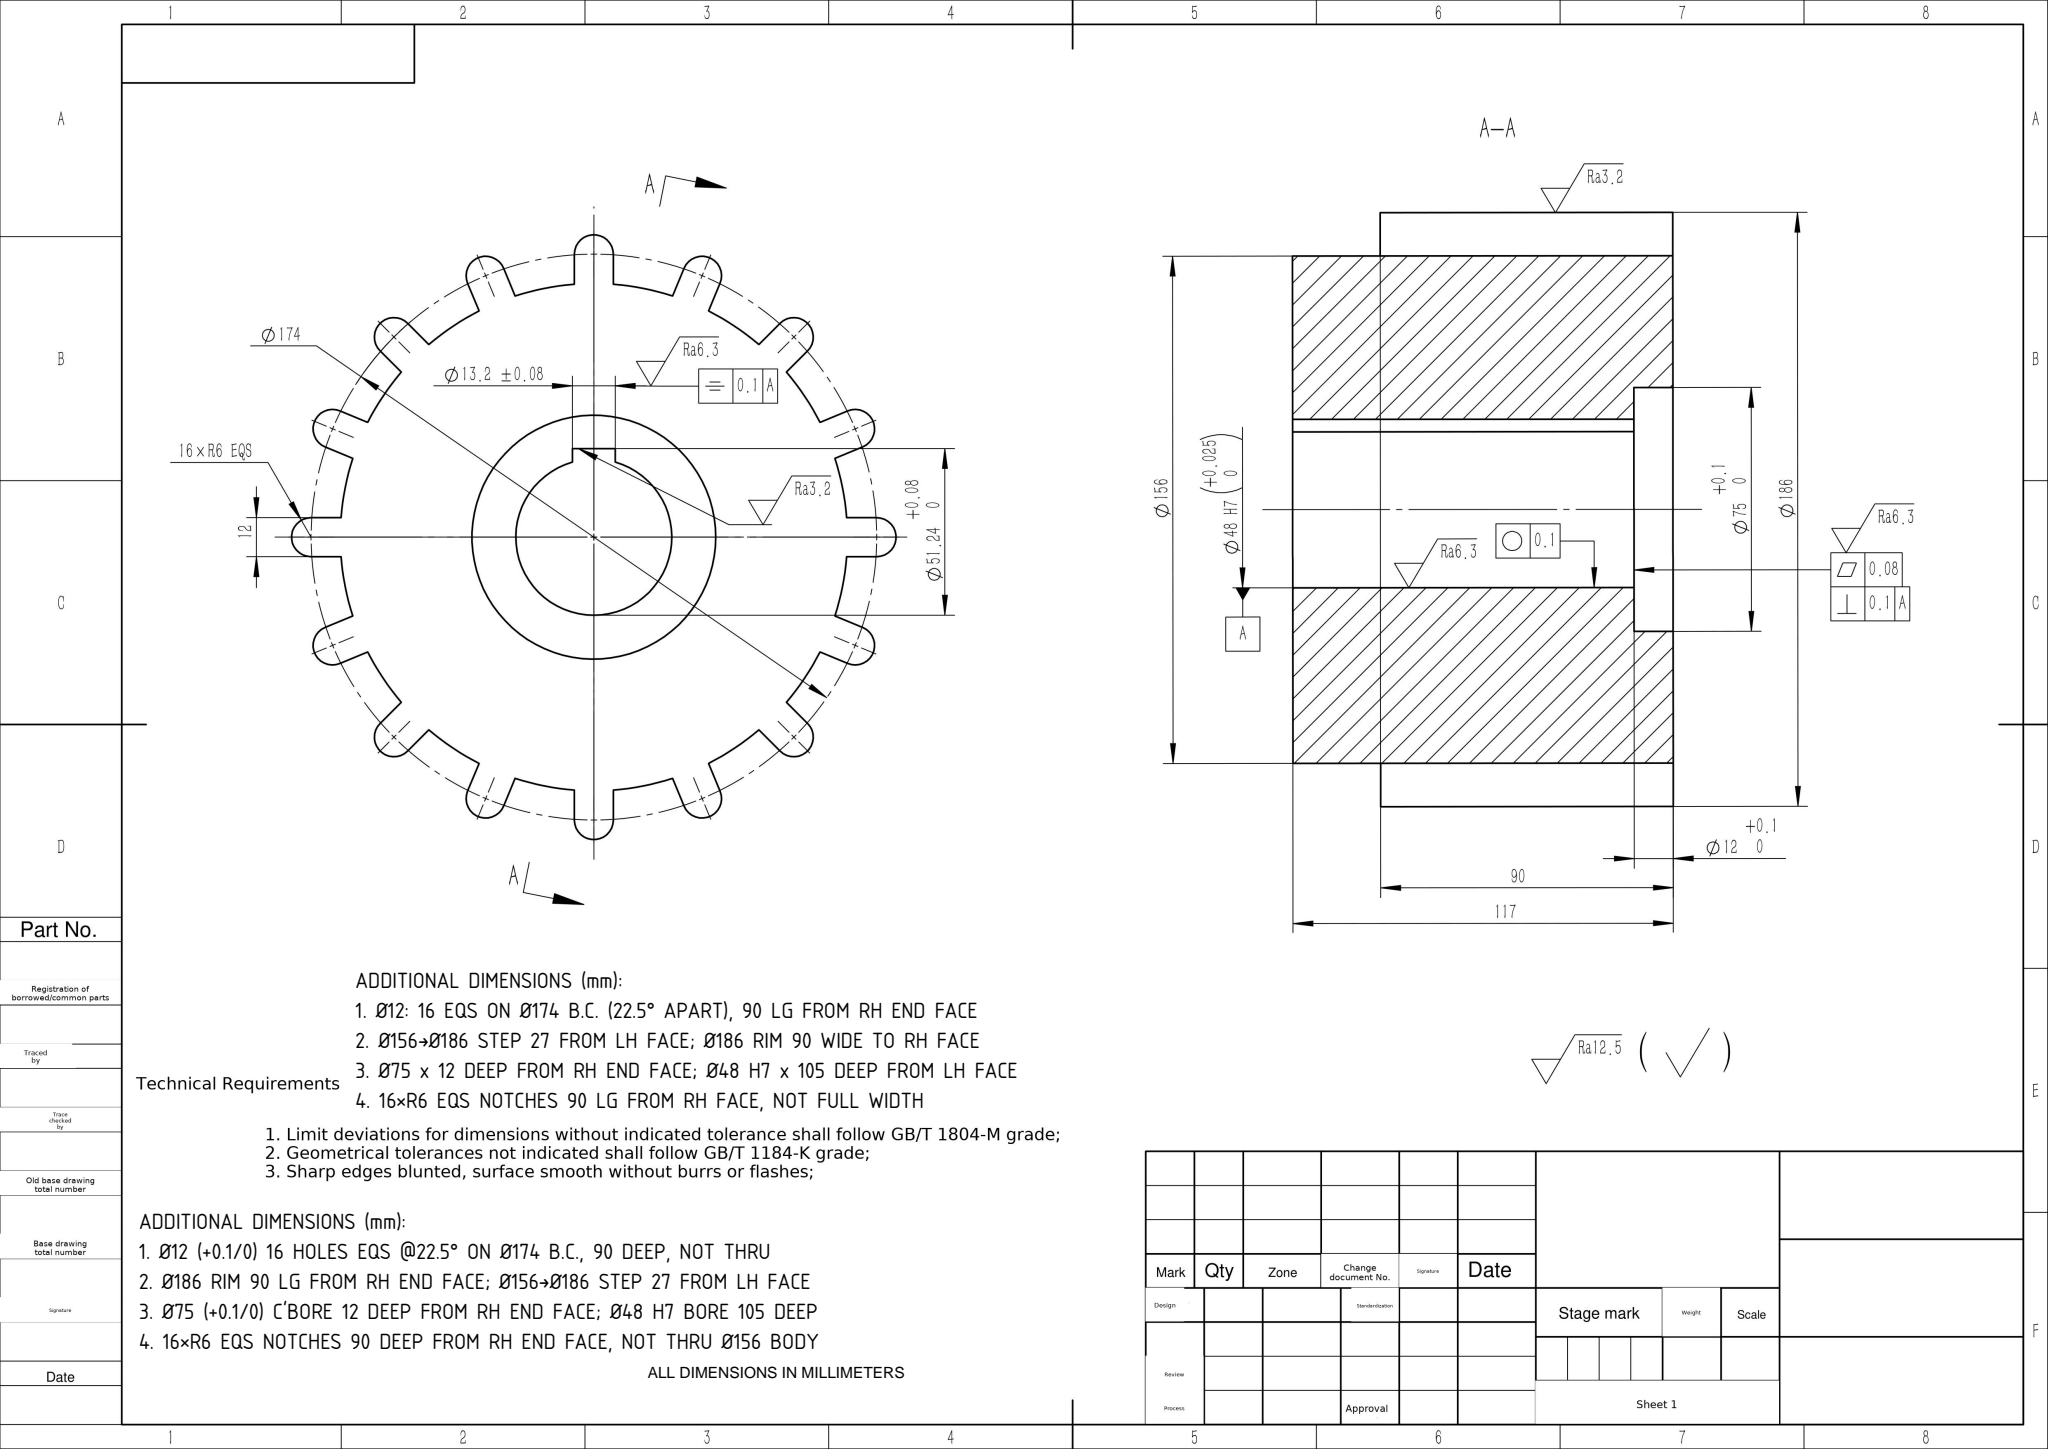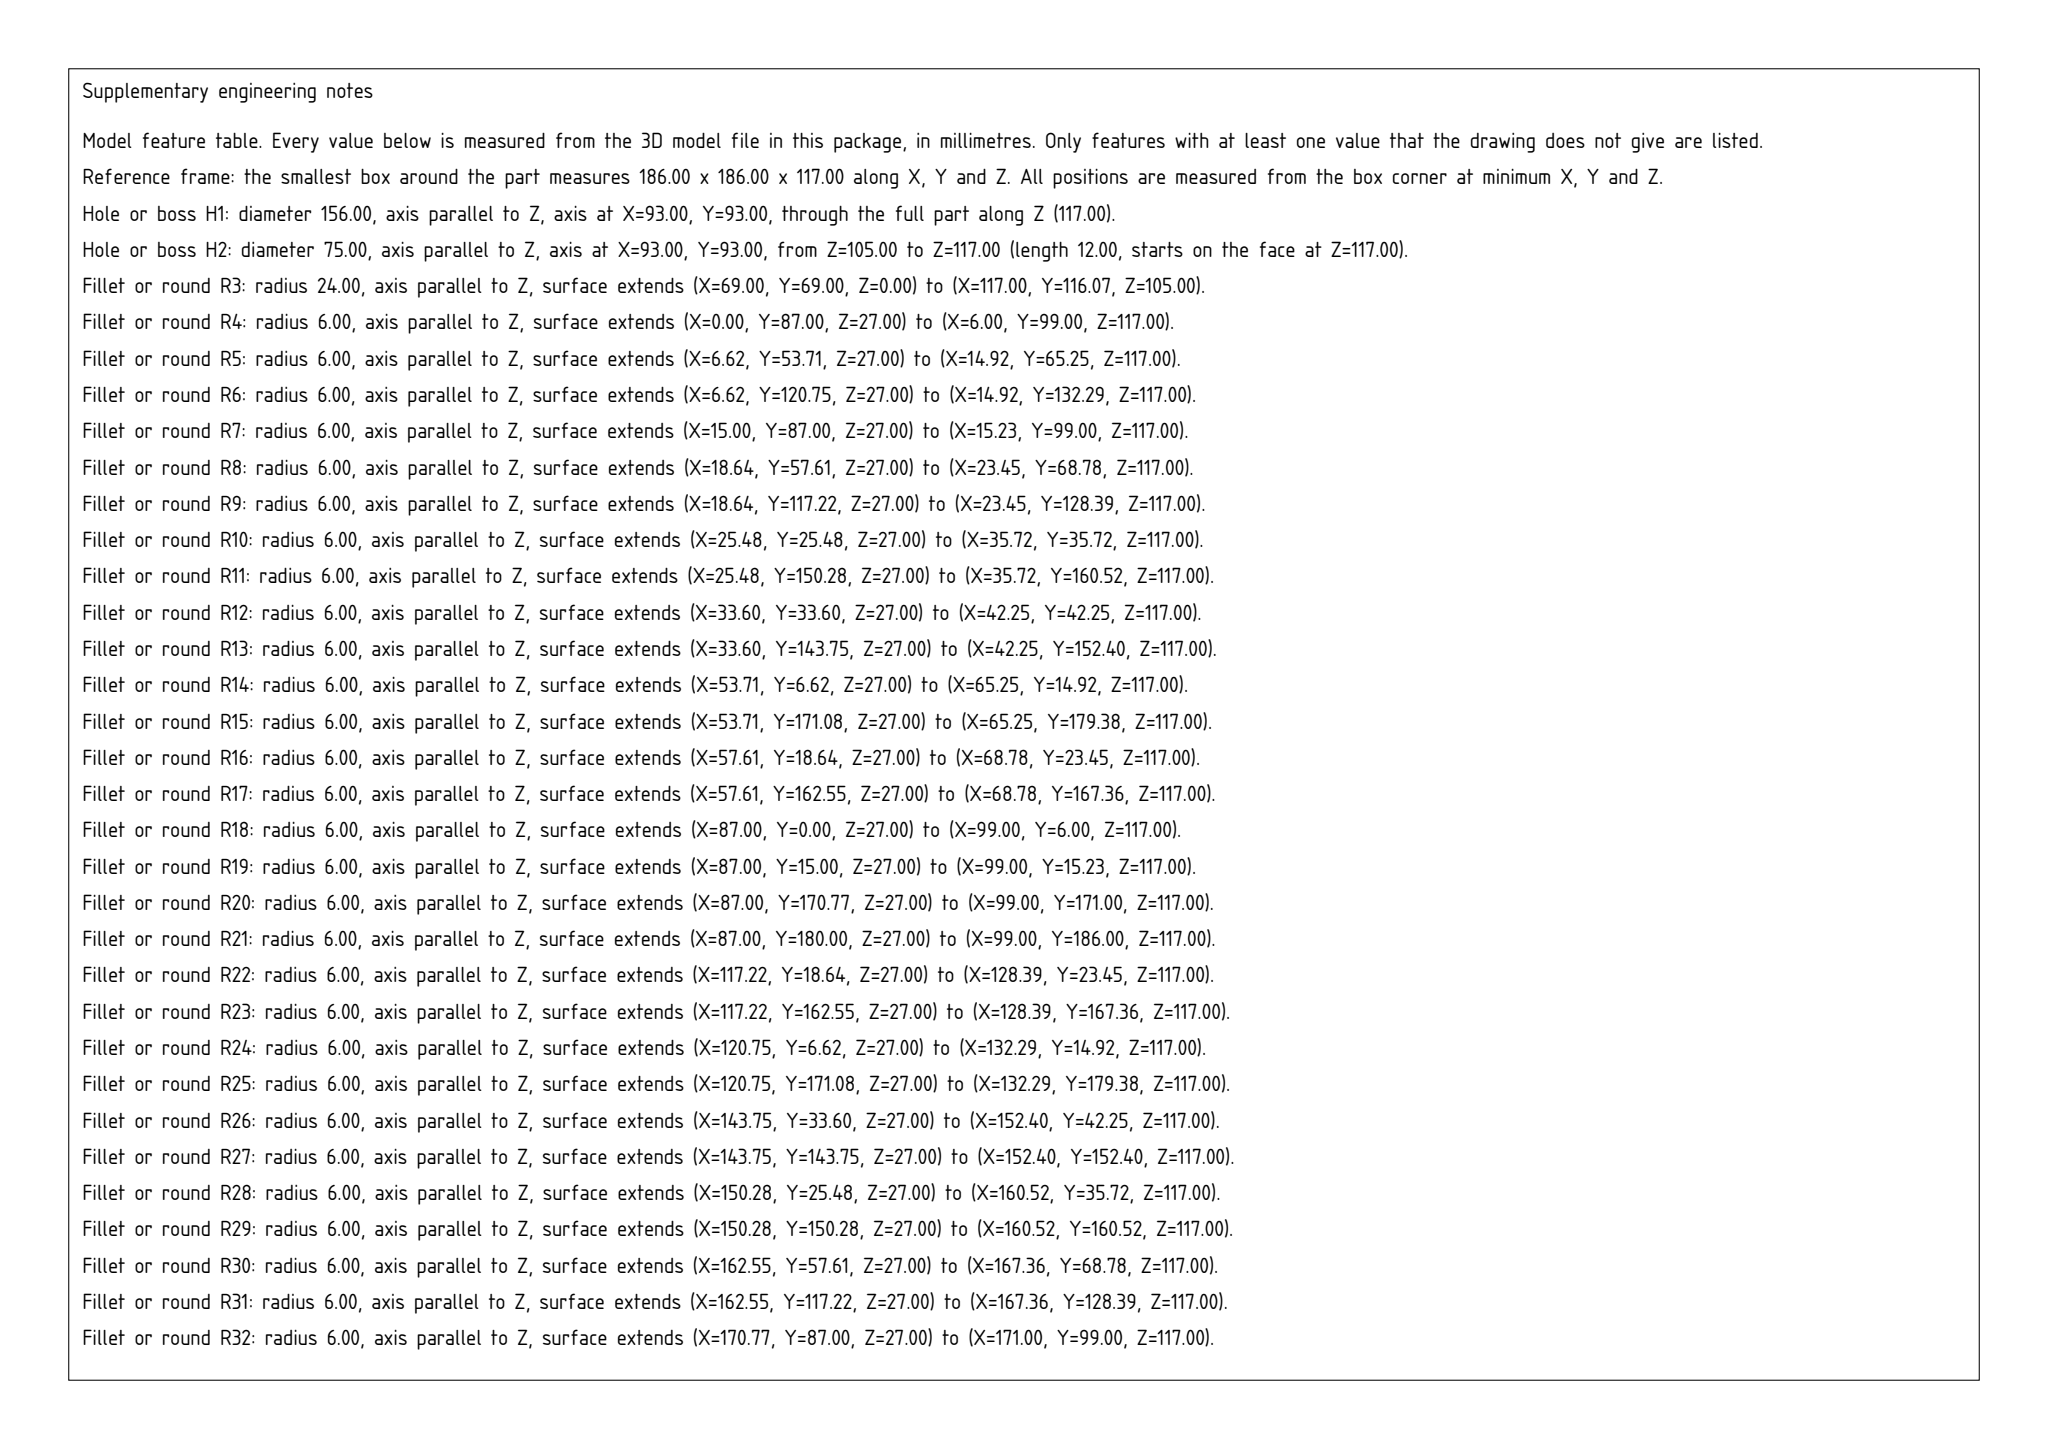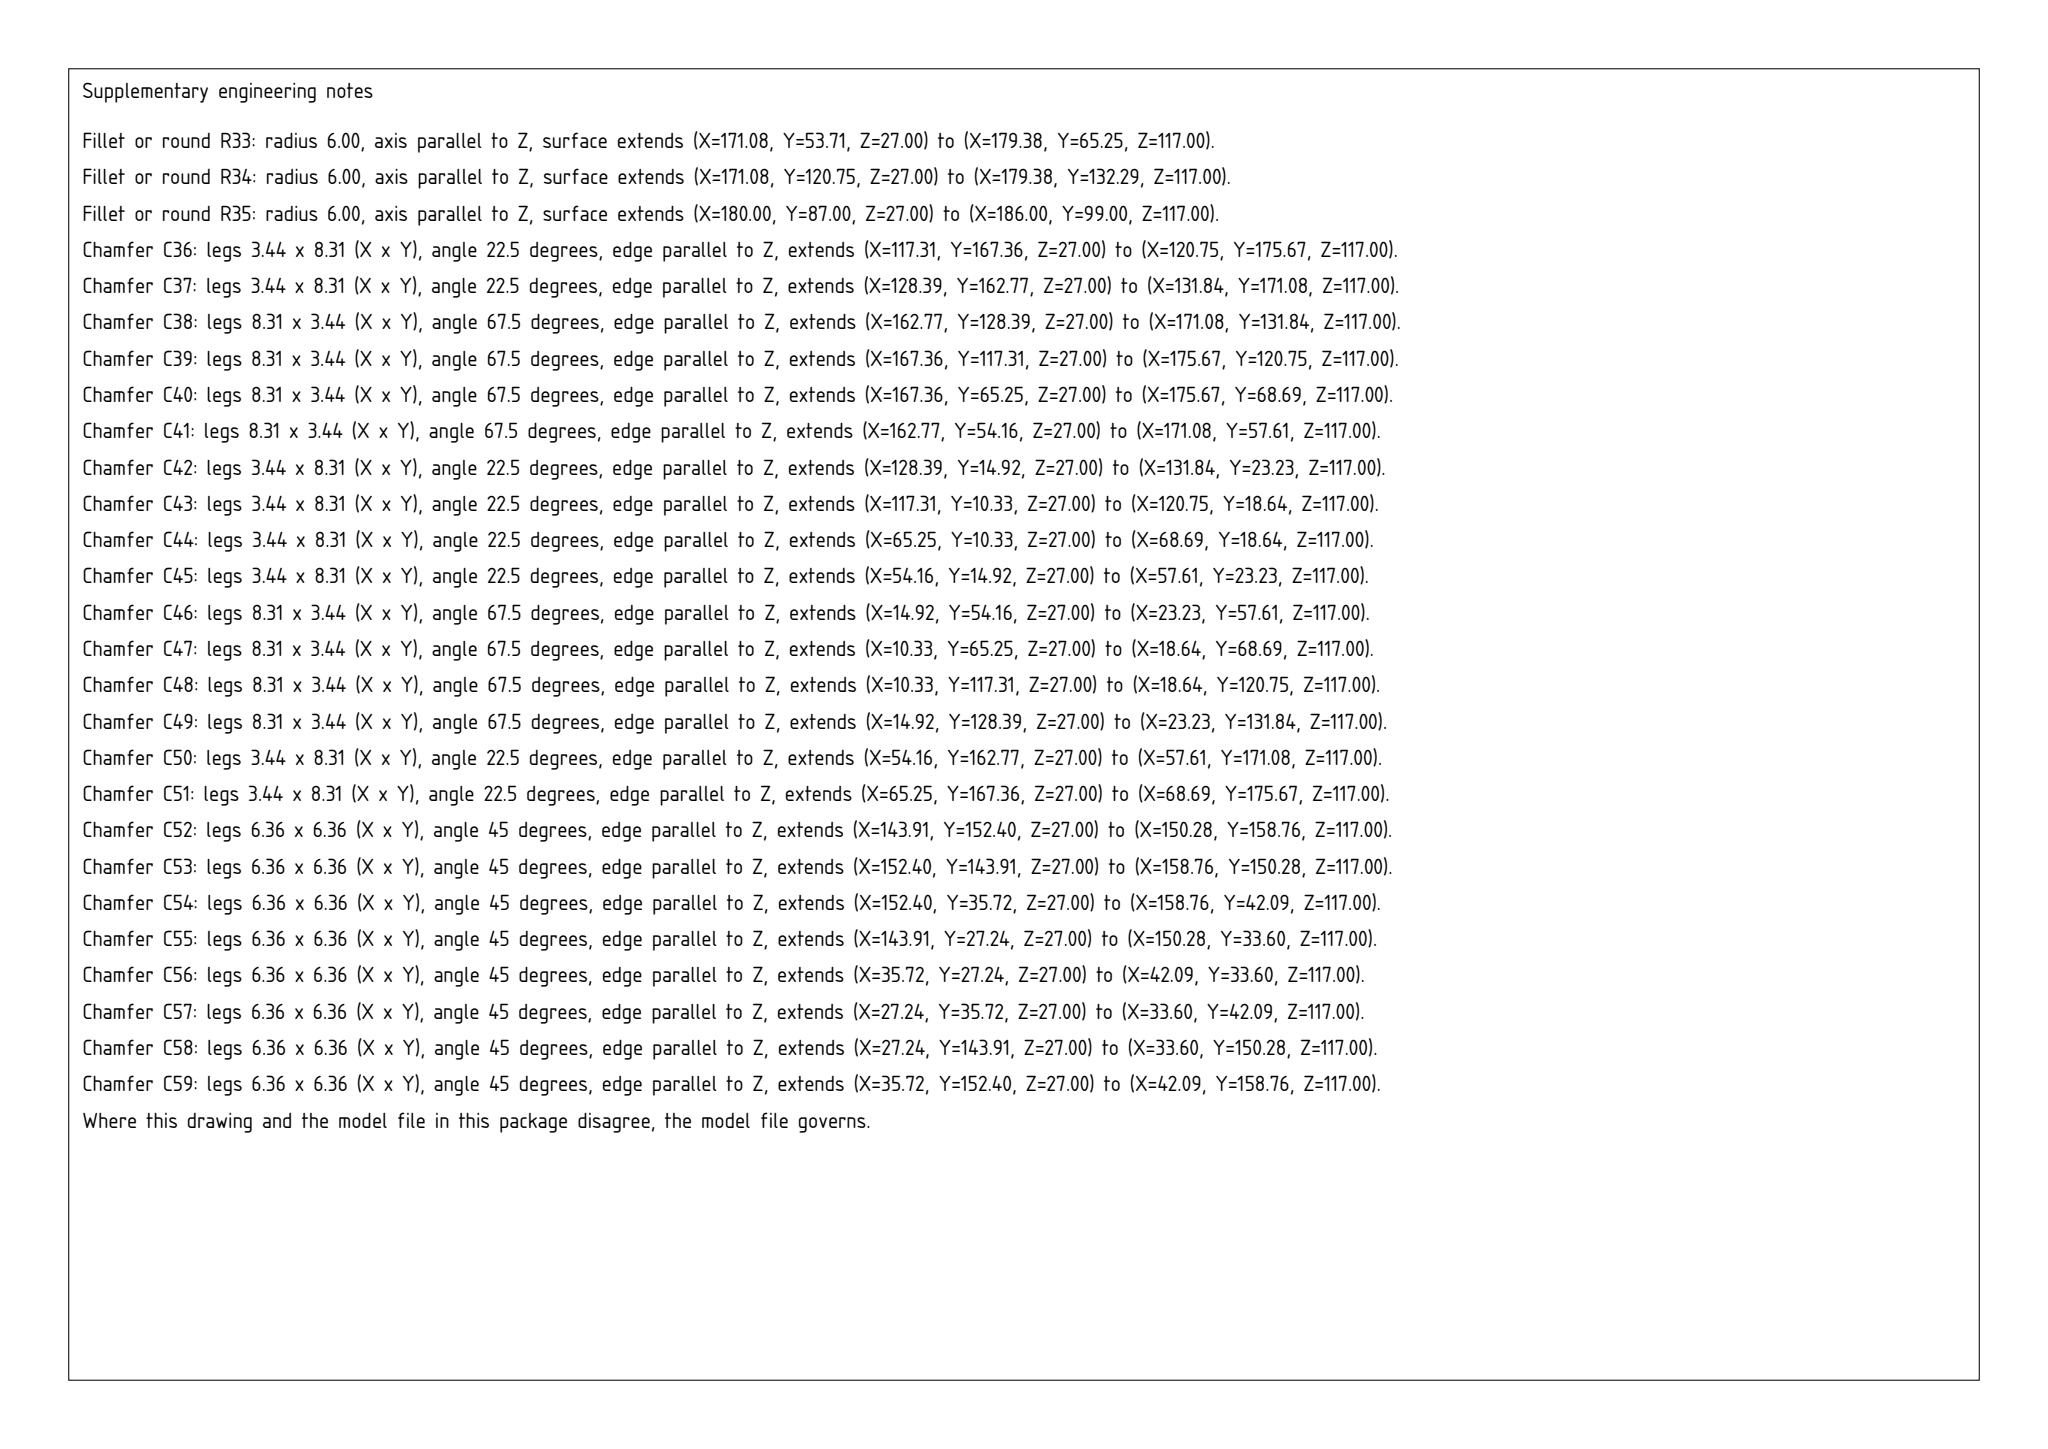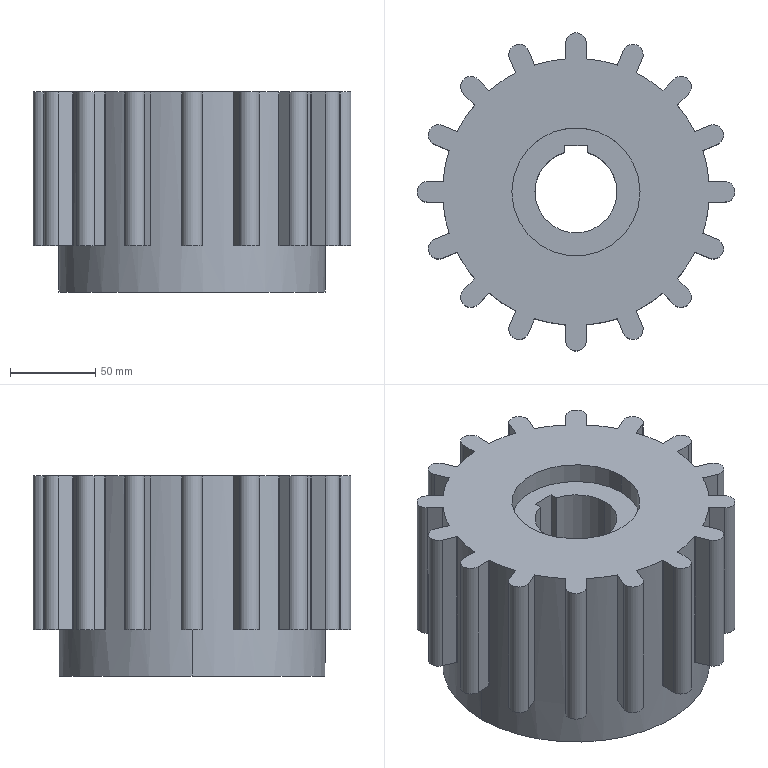Part | SolidWorks | mm | 1 solid | 116 faces | box 186 x 186 x 117 mm | volume 2226620 mm3 | cylinder 62 | plane 54 | commonest cylinder face diameters 12 x55 48 x3 75 x2 156 x2